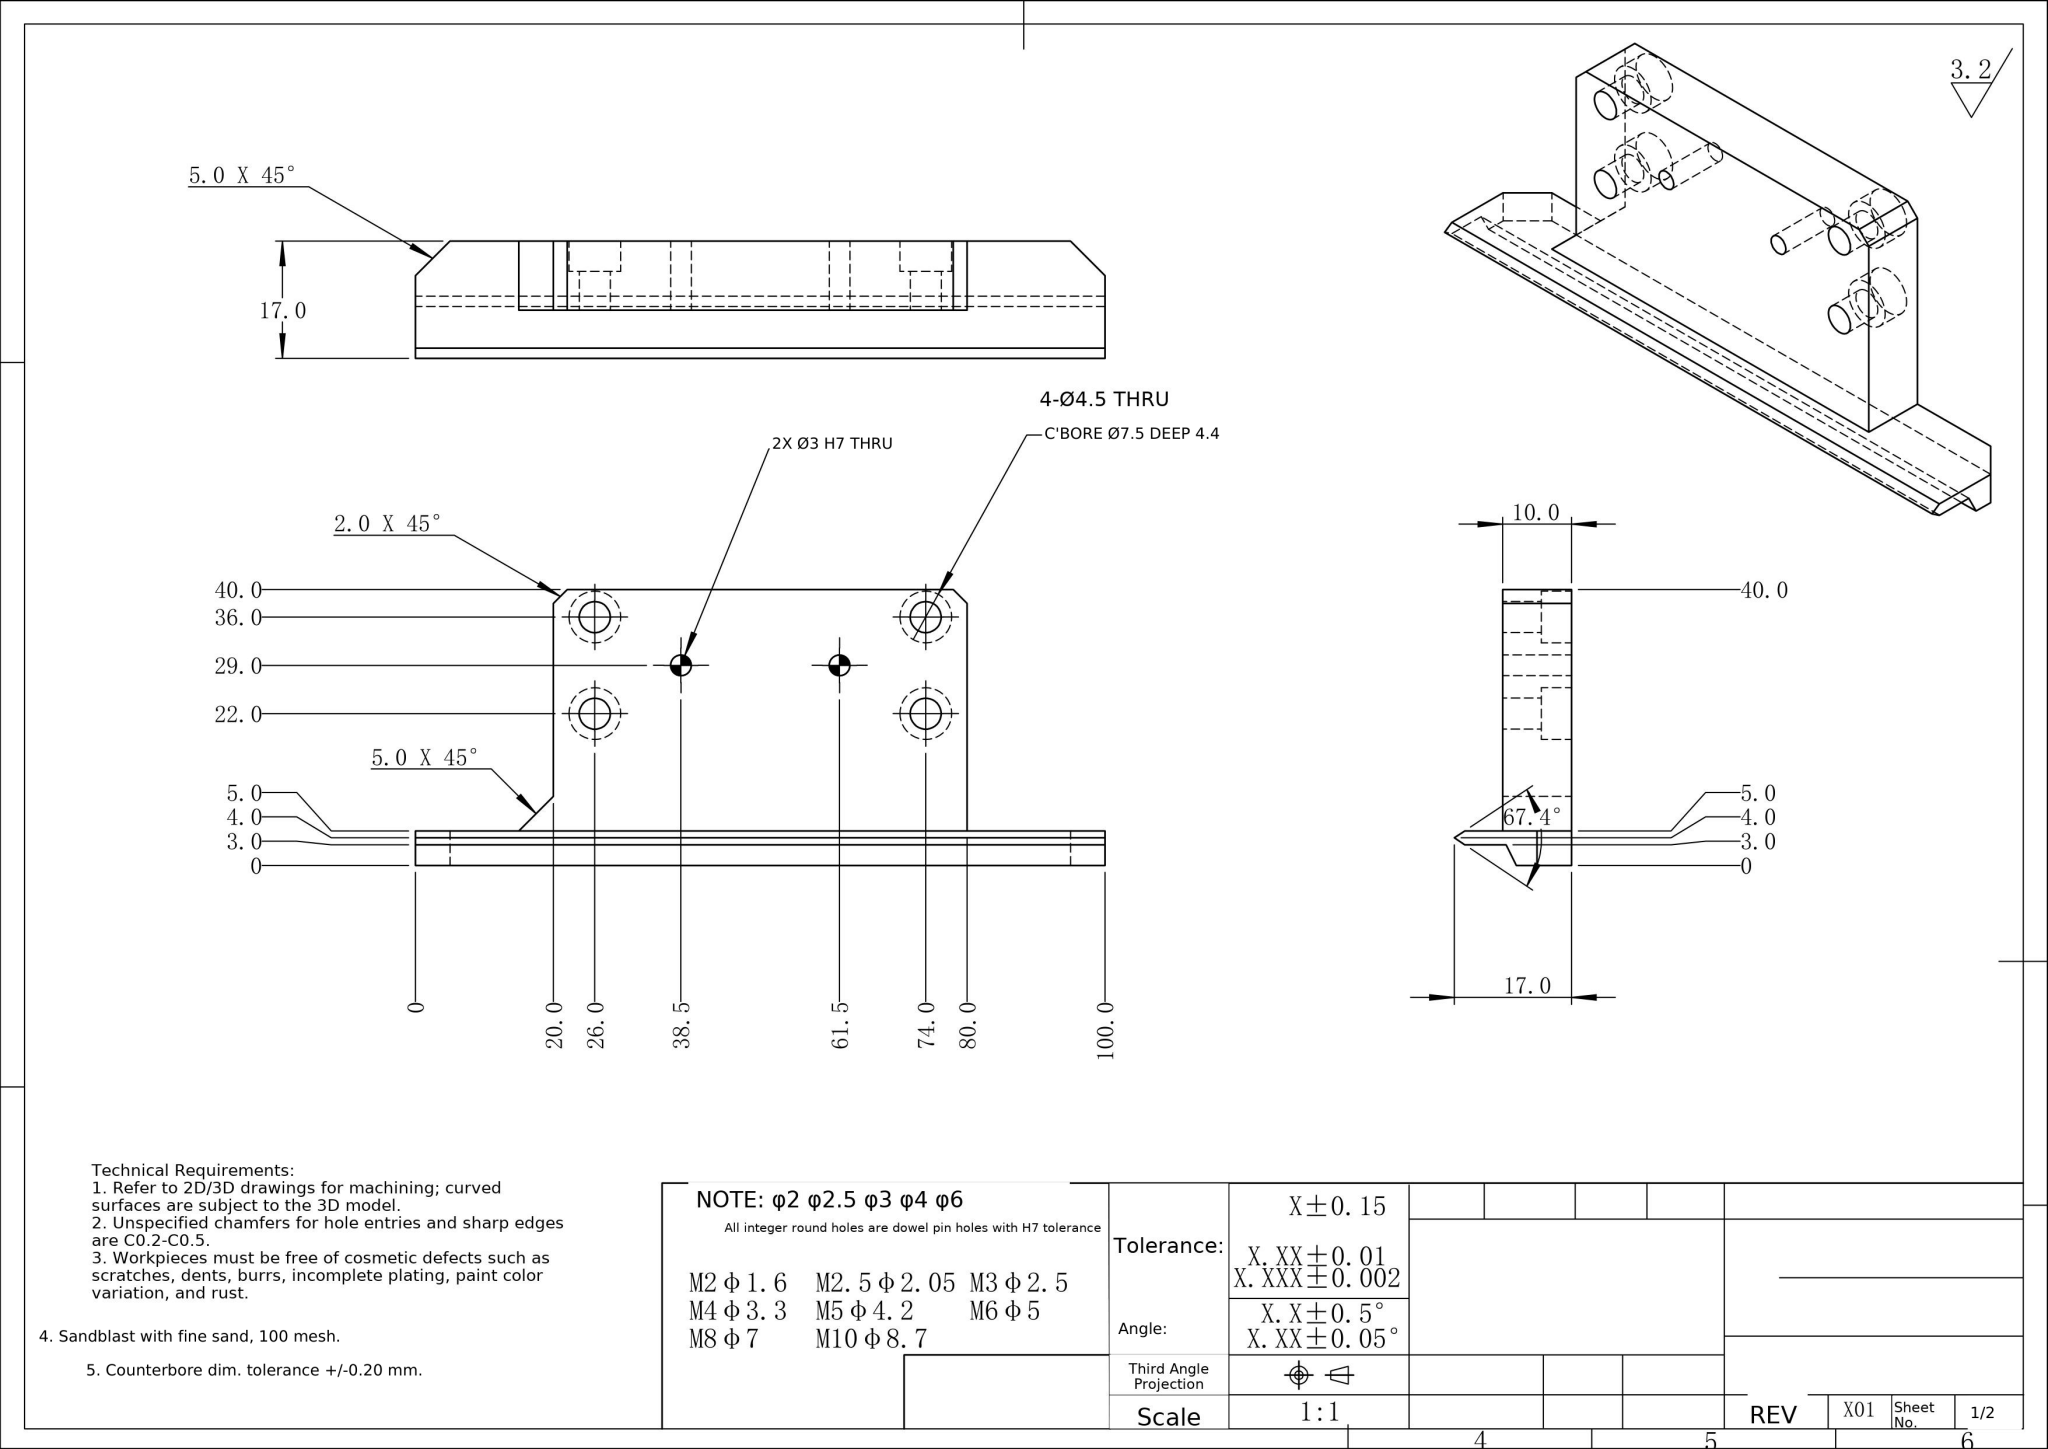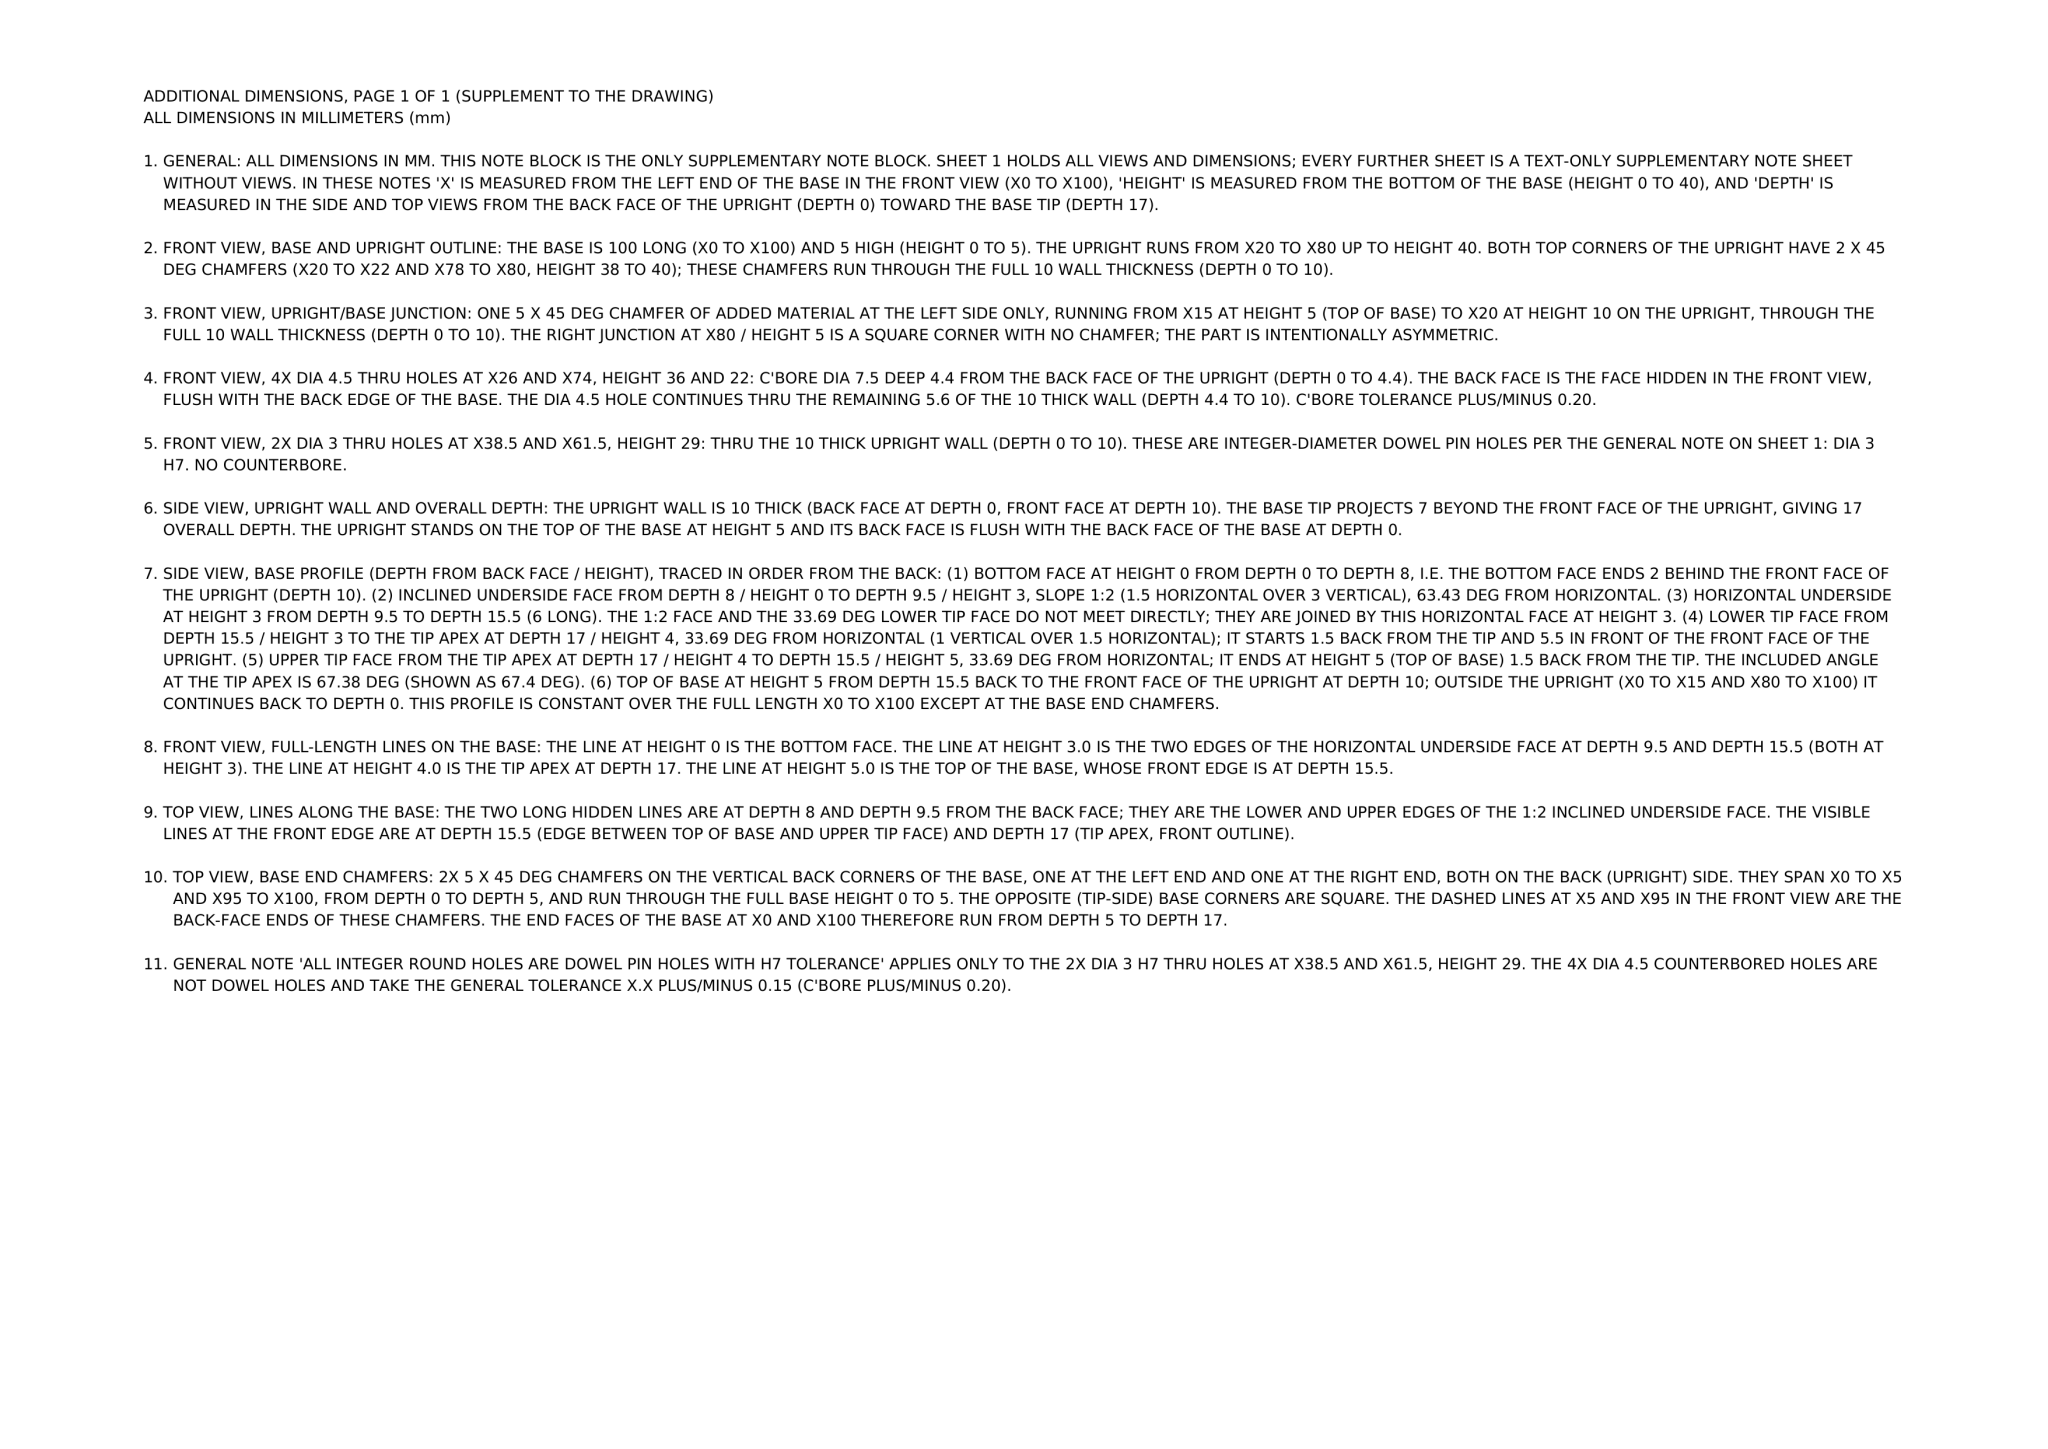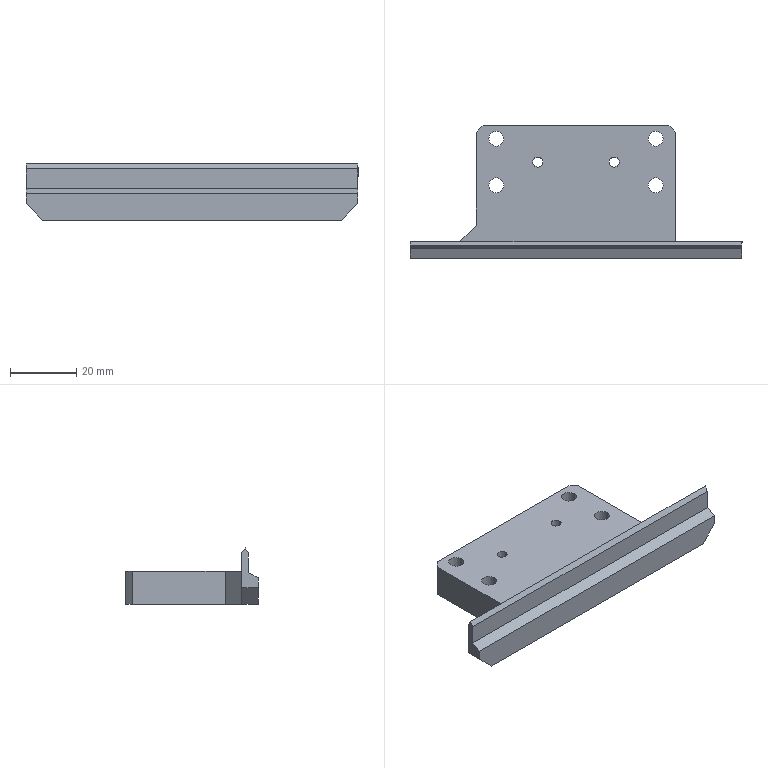Part | NX | mm | 1 solid | 42 faces | box 100 x 40 x 17 mm | volume 25560 mm3 | plane 22 | cylinder 20 | commonest cylinder face diameters 7.5 x8 4.5 x8 3 x4